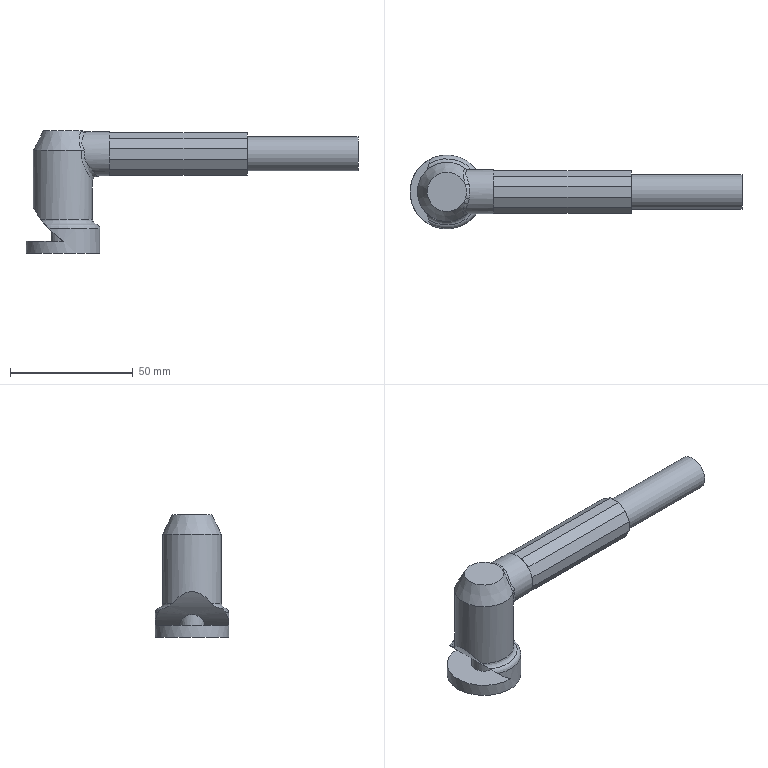Component | NX | PNEUM_GRINDER_PEN | 1 solid | 33 faces | volume 45098 mm3 | plane 19 | cylinder 7 | spline 4 | torus 2 | cone 1 | commonest cylinder face diameters 18 x1 14 x1 24 x1 78.138 x1 30 x1 10 x1 6 x1